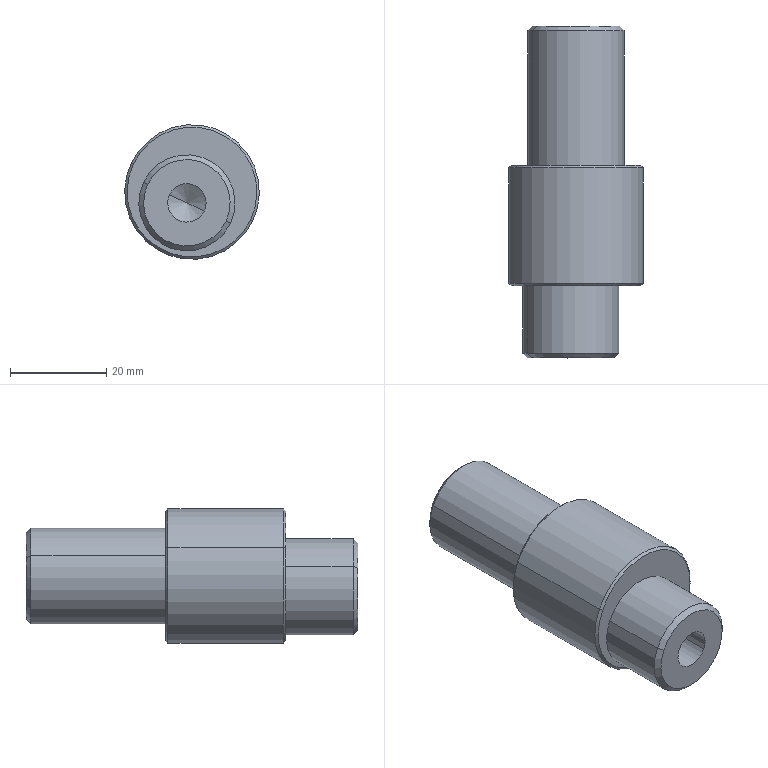Component | SolidWorks | Yk1.5.3RollerEccentricAxis-1 | 1 solid | 26 faces | box 28 x 69 x 28 mm | volume 27295 mm3 | cone 12 | cylinder 10 | plane 4 | commonest cylinder face diameters 8 x4 20 x4 28 x2 | material 45
build123d program:
from build123d import *

# Parameters (mm, degrees)
M8_TAPPED_HOLE2_D     = 8
M8_TAPPED_HOLE2_DEPTH = 15
M8_TAPPED_HOLE2_TIP   = 2.403
SKETCH4_R             = 10
BOSS_EXTRUDE1_DEPTH   = 15
CHAMFER1_SIZE         = 1
M8_TAPPED_HOLE1_D     = 8
M8_TAPPED_HOLE1_DEPTH = 20
M8_TAPPED_HOLE1_TIP   = 2.403
CHAMFER2_SIZE         = 0.5


with BuildPart() as part:
    # Sketch1 → Revolve1 (revolve)
    with BuildSketch(Plane.XY, mode=Mode.PRIVATE) as revolve1_sk:
        Polygon((14, 32.214), (0, 32.214), (0, 86.214), (10, 86.214), (10, 57.214), (14, 57.214), align=None)
    revolve(revolve1_sk.sketch.rotate(Axis((0, 0, 0), (0, 1, 0)), 90), axis=Axis((0, 0, 0), (0, 1, 0)))

    # M8 Tapped Hole2
    with Locations(Plane(origin=(0, 86.214, 0), x_dir=(1, 0, 0), z_dir=(0, 1, 0))):
        with Locations((0, 0)):
            Hole(M8_TAPPED_HOLE2_D / 2, depth=M8_TAPPED_HOLE2_DEPTH)
            with Locations((0, 0, -(M8_TAPPED_HOLE2_DEPTH + M8_TAPPED_HOLE2_TIP / 2))):  # 118° drill point
                Cone(0, M8_TAPPED_HOLE2_D / 2, M8_TAPPED_HOLE2_TIP, mode=Mode.SUBTRACT)

    # Sketch4 → Boss-Extrude1 (add)
    with BuildSketch(Plane(origin=(0, 32.214, 0), x_dir=(-1, 0, 0), z_dir=(0, -1, 0))):
        with Locations(Location((-2.5, 0, 0), (0, 0, 90))):
            Circle(SKETCH4_R)
    extrude(amount=BOSS_EXTRUDE1_DEPTH)

    # Chamfer1
    chamfer1_edges = [part.edges().sort_by_distance(p)[0] for p in [
        (2.5, 17.214, 10),
        (0, 86.214, 10),
    ]]
    chamfer(chamfer1_edges, length=CHAMFER1_SIZE)

    # M8 Tapped Hole1
    with Locations(Plane(origin=(0, 17.214, 0), x_dir=(-1, 0, 0), z_dir=(0, -1, 0))):
        with Locations((-2.5, 0)):
            Hole(M8_TAPPED_HOLE1_D / 2, depth=M8_TAPPED_HOLE1_DEPTH)
            with Locations((0, 0, -(M8_TAPPED_HOLE1_DEPTH + M8_TAPPED_HOLE1_TIP / 2))):  # 118° drill point
                Cone(0, M8_TAPPED_HOLE1_D / 2, M8_TAPPED_HOLE1_TIP, mode=Mode.SUBTRACT)

    # Chamfer2
    chamfer2_edges = [part.edges().sort_by_distance(p)[0] for p in [
        (0, 32.214, 14),
        (0, 57.214, 14),
    ]]
    chamfer(chamfer2_edges, length=CHAMFER2_SIZE)


solid = part.part

# Placed as in the assembly
solid = solid.moved(Location((-40.006, -57.214, 26), (180, 64.768, -180)))
STEP:
#1=COLOUR_RGB('',0.7922,0.8196,0.9333);
#2=FILL_AREA_STYLE_COLOUR('',#1);
#3=FILL_AREA_STYLE('',(#2));
#4=SURFACE_STYLE_FILL_AREA(#3);
#5=SURFACE_SIDE_STYLE('',(#4));
#6=SURFACE_STYLE_USAGE(.BOTH.,#5);
#7=PRESENTATION_STYLE_ASSIGNMENT((#6));
#8=CARTESIAN_POINT('',(-1.094,-0.,0.7971));
#9=VERTEX_POINT('',#8);
#10=CARTESIAN_POINT('',(-2.056,-0.,1.25));
#11=VERTEX_POINT('',#10);
#12=CARTESIAN_POINT('',(-1.575,-0.,1.024));
#13=DIRECTION('',(0.,1.,0.));
#14=DIRECTION('',(0.9046,0.,-0.4263));
#15=AXIS2_PLACEMENT_3D('',#12,#13,#14);
#16=CIRCLE('',#15,0.5315);
#17=EDGE_CURVE('',#9,#11,#16,.T.);
#18=ORIENTED_EDGE('',*,*,#17,.F.);
#19=CARTESIAN_POINT('',(-1.076,-0.01969,0.7887));
#20=VERTEX_POINT('',#19);
#21=CARTESIAN_POINT('',(-1.076,-0.01969,0.7887));
#22=DIRECTION('',(0.6396,-0.7071,-0.3014));
#23=VECTOR('',#22,39.37);
#24=LINE('',#21,#23);
#25=EDGE_CURVE('',#9,#20,#24,.T.);
#26=ORIENTED_EDGE('',*,*,#25,.T.);
#27=CARTESIAN_POINT('',(-2.074,-0.01969,1.259));
#28=VERTEX_POINT('',#27);
#29=CARTESIAN_POINT('',(-1.575,-0.01969,1.024));
#30=DIRECTION('',(0.,-1.,0.));
#31=DIRECTION('',(0.9046,0.,-0.4263));
#32=AXIS2_PLACEMENT_3D('',#29,#30,#31);
#33=CIRCLE('',#32,0.5512);
#34=EDGE_CURVE('',#28,#20,#33,.T.);
#35=ORIENTED_EDGE('',*,*,#34,.F.);
#36=CARTESIAN_POINT('',(-2.074,-0.01969,1.259));
#37=DIRECTION('',(-0.6396,-0.7071,0.3014));
#38=VECTOR('',#37,39.37);
#39=LINE('',#36,#38);
#40=EDGE_CURVE('',#11,#28,#39,.T.);
#41=ORIENTED_EDGE('',*,*,#40,.F.);
#42=EDGE_LOOP('',(#18,#26,#35,#41));
#43=FACE_OUTER_BOUND('',#42,.T.);
#44=CARTESIAN_POINT('',(-1.575,-0.01969,1.024));
#45=DIRECTION('',(0.,-1.,0.));
#46=DIRECTION('',(-0.9046,0.,0.4263));
#47=AXIS2_PLACEMENT_3D('',#44,#45,#46);
#48=CONICAL_SURFACE('',#47,0.5512,0.7854);
#49=ADVANCED_FACE('',(#43),#48,.T.);
#50=CARTESIAN_POINT('',(-2.056,-0.9843,1.25));
#51=VERTEX_POINT('',#50);
#52=CARTESIAN_POINT('',(-1.094,-0.9843,0.7971));
#53=VERTEX_POINT('',#52);
#54=CARTESIAN_POINT('',(-1.575,-0.9843,1.024));
#55=DIRECTION('',(0.,-1.,0.));
#56=DIRECTION('',(-0.9046,0.,0.4263));
#57=AXIS2_PLACEMENT_3D('',#54,#55,#56);
#58=CIRCLE('',#57,0.5315);
#59=EDGE_CURVE('',#51,#53,#58,.T.);
#60=ORIENTED_EDGE('',*,*,#59,.F.);
#61=CARTESIAN_POINT('',(-2.074,-0.9646,1.259));
#62=VERTEX_POINT('',#61);
#63=CARTESIAN_POINT('',(-2.056,-0.9843,1.25));
#64=DIRECTION('',(-0.6396,0.7071,0.3014));
#65=VECTOR('',#64,39.37);
#66=LINE('',#63,#65);
#67=EDGE_CURVE('',#51,#62,#66,.T.);
#68=ORIENTED_EDGE('',*,*,#67,.T.);
#69=CARTESIAN_POINT('',(-1.076,-0.9646,0.7887));
#70=VERTEX_POINT('',#69);
#71=CARTESIAN_POINT('',(-1.575,-0.9646,1.024));
#72=DIRECTION('',(0.,1.,0.));
#73=DIRECTION('',(-0.9046,0.,0.4263));
#74=AXIS2_PLACEMENT_3D('',#71,#72,#73);
#75=CIRCLE('',#74,0.5512);
#76=EDGE_CURVE('',#70,#62,#75,.T.);
#77=ORIENTED_EDGE('',*,*,#76,.F.);
#78=CARTESIAN_POINT('',(-1.094,-0.9843,0.7971));
#79=DIRECTION('',(0.6396,0.7071,-0.3014));
#80=VECTOR('',#79,39.37);
#81=LINE('',#78,#80);
#82=EDGE_CURVE('',#53,#70,#81,.T.);
#83=ORIENTED_EDGE('',*,*,#82,.F.);
#84=EDGE_LOOP('',(#60,#68,#77,#83));
#85=FACE_OUTER_BOUND('',#84,.T.);
#86=CARTESIAN_POINT('',(-1.575,-0.9843,1.024));
#87=DIRECTION('',(0.,1.,0.));
#88=DIRECTION('',(0.9046,0.,-0.4263));
#89=AXIS2_PLACEMENT_3D('',#86,#87,#88);
#90=CONICAL_SURFACE('',#89,0.5315,0.7854);
#91=ADVANCED_FACE('',(#85),#90,.T.);
#92=CARTESIAN_POINT('',(-1.475,-0.7874,0.8675));
#93=VERTEX_POINT('',#92);
#94=CARTESIAN_POINT('',(-1.759,-0.7874,1.002));
#95=VERTEX_POINT('',#94);
#96=CARTESIAN_POINT('',(-1.617,-0.7874,0.9346));
#97=DIRECTION('',(0.,-1.,0.));
#98=DIRECTION('',(-0.9046,0.,0.4263));
#99=AXIS2_PLACEMENT_3D('',#96,#97,#98);
#100=CIRCLE('',#99,0.1575);
#101=EDGE_CURVE('',#93,#95,#100,.T.);
#102=ORIENTED_EDGE('',*,*,#101,.F.);
#103=CARTESIAN_POINT('',(-1.475,-1.575,0.8675));
#104=VERTEX_POINT('',#103);
#105=CARTESIAN_POINT('',(-1.475,-1.575,0.8675));
#106=DIRECTION('',(0.,-1.,0.));
#107=VECTOR('',#106,39.37);
#108=LINE('',#105,#107);
#109=EDGE_CURVE('',#93,#104,#108,.T.);
#110=ORIENTED_EDGE('',*,*,#109,.T.);
#111=CARTESIAN_POINT('',(-1.759,-1.575,1.002));
#112=VERTEX_POINT('',#111);
#113=CARTESIAN_POINT('',(-1.617,-1.575,0.9346));
#114=DIRECTION('',(0.,-1.,0.));
#115=DIRECTION('',(-0.9046,0.,0.4263));
#116=AXIS2_PLACEMENT_3D('',#113,#114,#115);
#117=CIRCLE('',#116,0.1575);
#118=EDGE_CURVE('',#104,#112,#117,.T.);
#119=ORIENTED_EDGE('',*,*,#118,.T.);
#120=CARTESIAN_POINT('',(-1.759,-1.575,1.002));
#121=DIRECTION('',(0.,-1.,0.));
#122=VECTOR('',#121,39.37);
#123=LINE('',#120,#122);
#124=EDGE_CURVE('',#95,#112,#123,.T.);
#125=ORIENTED_EDGE('',*,*,#124,.F.);
#126=EDGE_LOOP('',(#102,#110,#119,#125));
#127=FACE_OUTER_BOUND('',#126,.T.);
#128=CARTESIAN_POINT('',(-1.617,-1.575,0.9346));
#129=DIRECTION('',(0.,-1.,0.));
#130=DIRECTION('',(-0.9046,0.,0.4263));
#131=AXIS2_PLACEMENT_3D('',#128,#129,#130);
#132=CYLINDRICAL_SURFACE('',#131,0.1575);
#133=ADVANCED_FACE('',(#127),#132,.F.);
#134=CARTESIAN_POINT('',(-1.617,-0.6928,0.9346));
#135=VERTEX_POINT('',#134);
#136=CARTESIAN_POINT('',(-1.759,-0.7874,1.002));
#137=DIRECTION('',(-0.7754,-0.515,0.3654));
#138=VECTOR('',#137,39.37);
#139=LINE('',#136,#138);
#140=EDGE_CURVE('',#135,#95,#139,.T.);
#141=ORIENTED_EDGE('',*,*,#140,.F.);
#142=CARTESIAN_POINT('',(-1.475,-0.7874,0.8675));
#143=DIRECTION('',(0.7754,-0.515,-0.3654));
#144=VECTOR('',#143,39.37);
#145=LINE('',#142,#144);
#146=EDGE_CURVE('',#135,#93,#145,.T.);
#147=ORIENTED_EDGE('',*,*,#146,.T.);
#148=ORIENTED_EDGE('',*,*,#101,.T.);
#149=EDGE_LOOP('',(#141,#147,#148));
#150=FACE_OUTER_BOUND('',#149,.T.);
#151=CARTESIAN_POINT('',(-1.617,-0.7874,0.9346));
#152=DIRECTION('',(0.,-1.,0.));
#153=DIRECTION('',(-0.9046,0.,0.4263));
#154=AXIS2_PLACEMENT_3D('',#151,#152,#153);
#155=CONICAL_SURFACE('',#154,0.1575,1.03);
#156=ADVANCED_FACE('',(#150),#155,.F.);
#157=CARTESIAN_POINT('',(-1.255,1.142,0.8726));
#158=VERTEX_POINT('',#157);
#159=CARTESIAN_POINT('',(-1.896,1.142,1.175));
#160=VERTEX_POINT('',#159);
#161=CARTESIAN_POINT('',(-1.575,1.142,1.024));
#162=DIRECTION('',(0.,1.,0.));
#163=DIRECTION('',(0.9046,0.,-0.4263));
#164=AXIS2_PLACEMENT_3D('',#161,#162,#163);
#165=CIRCLE('',#164,0.3543);
#166=EDGE_CURVE('',#158,#160,#165,.T.);
#167=ORIENTED_EDGE('',*,*,#166,.F.);
#168=CARTESIAN_POINT('',(-1.219,1.102,0.8558));
#169=VERTEX_POINT('',#168);
#170=CARTESIAN_POINT('',(-1.219,1.102,0.8558));
#171=DIRECTION('',(0.6396,-0.7071,-0.3014));
#172=VECTOR('',#171,39.37);
#173=LINE('',#170,#172);
#174=EDGE_CURVE('',#158,#169,#173,.T.);
#175=ORIENTED_EDGE('',*,*,#174,.T.);
#176=CARTESIAN_POINT('',(-1.931,1.102,1.191));
#177=VERTEX_POINT('',#176);
#178=CARTESIAN_POINT('',(-1.575,1.102,1.024));
#179=DIRECTION('',(0.,-1.,0.));
#180=DIRECTION('',(0.9046,0.,-0.4263));
#181=AXIS2_PLACEMENT_3D('',#178,#179,#180);
#182=CIRCLE('',#181,0.3937);
#183=EDGE_CURVE('',#177,#169,#182,.T.);
#184=ORIENTED_EDGE('',*,*,#183,.F.);
#185=CARTESIAN_POINT('',(-1.931,1.102,1.191));
#186=DIRECTION('',(-0.6396,-0.7071,0.3014));
#187=VECTOR('',#186,39.37);
#188=LINE('',#185,#187);
#189=EDGE_CURVE('',#160,#177,#188,.T.);
#190=ORIENTED_EDGE('',*,*,#189,.F.);
#191=EDGE_LOOP('',(#167,#175,#184,#190));
#192=FACE_OUTER_BOUND('',#191,.T.);
#193=CARTESIAN_POINT('',(-1.575,1.102,1.024));
#194=DIRECTION('',(0.,-1.,0.));
#195=DIRECTION('',(-0.9046,0.,0.4263));
#196=AXIS2_PLACEMENT_3D('',#193,#194,#195);
#197=CONICAL_SURFACE('',#196,0.3937,0.7854);
#198=ADVANCED_FACE('',(#192),#197,.T.);
#199=CARTESIAN_POINT('',(-1.938,-1.575,1.086));
#200=VERTEX_POINT('',#199);
#201=CARTESIAN_POINT('',(-1.296,-1.575,0.7835));
#202=VERTEX_POINT('',#201);
#203=CARTESIAN_POINT('',(-1.617,-1.575,0.9346));
#204=DIRECTION('',(0.,-1.,0.));
#205=DIRECTION('',(-0.9046,0.,0.4263));
#206=AXIS2_PLACEMENT_3D('',#203,#204,#205);
#207=CIRCLE('',#206,0.3543);
#208=EDGE_CURVE('',#200,#202,#207,.T.);
#209=ORIENTED_EDGE('',*,*,#208,.F.);
#210=CARTESIAN_POINT('',(-1.973,-1.535,1.102));
#211=VERTEX_POINT('',#210);
#212=CARTESIAN_POINT('',(-1.938,-1.575,1.086));
#213=DIRECTION('',(-0.6396,0.7071,0.3014));
#214=VECTOR('',#213,39.37);
#215=LINE('',#212,#214);
#216=EDGE_CURVE('',#200,#211,#215,.T.);
#217=ORIENTED_EDGE('',*,*,#216,.T.);
#218=CARTESIAN_POINT('',(-1.261,-1.535,0.7668));
#219=VERTEX_POINT('',#218);
#220=CARTESIAN_POINT('',(-1.617,-1.535,0.9346));
#221=DIRECTION('',(0.,1.,0.));
#222=DIRECTION('',(-0.9046,0.,0.4263));
#223=AXIS2_PLACEMENT_3D('',#220,#221,#222);
#224=CIRCLE('',#223,0.3937);
#225=EDGE_CURVE('',#219,#211,#224,.T.);
#226=ORIENTED_EDGE('',*,*,#225,.F.);
#227=CARTESIAN_POINT('',(-1.296,-1.575,0.7835));
#228=DIRECTION('',(0.6396,0.7071,-0.3014));
#229=VECTOR('',#228,39.37);
#230=LINE('',#227,#229);
#231=EDGE_CURVE('',#202,#219,#230,.T.);
#232=ORIENTED_EDGE('',*,*,#231,.F.);
#233=EDGE_LOOP('',(#209,#217,#226,#232));
#234=FACE_OUTER_BOUND('',#233,.T.);
#235=CARTESIAN_POINT('',(-1.617,-1.575,0.9346));
#236=DIRECTION('',(0.,1.,0.));
#237=DIRECTION('',(0.9046,0.,-0.4263));
#238=AXIS2_PLACEMENT_3D('',#235,#236,#237);
#239=CONICAL_SURFACE('',#238,0.3543,0.7854);
#240=ADVANCED_FACE('',(#234),#239,.T.);
#241=ORIENTED_EDGE('',*,*,#225,.T.);
#242=CARTESIAN_POINT('',(-1.973,-0.9843,1.102));
#243=VERTEX_POINT('',#242);
#244=CARTESIAN_POINT('',(-1.973,-1.575,1.102));
#245=DIRECTION('',(0.,1.,0.));
#246=VECTOR('',#245,39.37);
#247=LINE('',#244,#246);
#248=EDGE_CURVE('',#211,#243,#247,.T.);
#249=ORIENTED_EDGE('',*,*,#248,.T.);
#250=CARTESIAN_POINT('',(-1.261,-0.9843,0.7668));
#251=VERTEX_POINT('',#250);
#252=CARTESIAN_POINT('',(-1.617,-0.9843,0.9346));
#253=DIRECTION('',(0.,-1.,0.));
#254=DIRECTION('',(-0.9046,0.,0.4263));
#255=AXIS2_PLACEMENT_3D('',#252,#253,#254);
#256=CIRCLE('',#255,0.3937);
#257=EDGE_CURVE('',#243,#251,#256,.T.);
#258=ORIENTED_EDGE('',*,*,#257,.T.);
#259=CARTESIAN_POINT('',(-1.261,-1.575,0.7668));
#260=DIRECTION('',(0.,1.,0.));
#261=VECTOR('',#260,39.37);
#262=LINE('',#259,#261);
#263=EDGE_CURVE('',#219,#251,#262,.T.);
#264=ORIENTED_EDGE('',*,*,#263,.F.);
#265=EDGE_LOOP('',(#241,#249,#258,#264));
#266=FACE_OUTER_BOUND('',#265,.T.);
#267=CARTESIAN_POINT('',(-1.617,-1.575,0.9346));
#268=DIRECTION('',(0.,1.,0.));
#269=DIRECTION('',(0.9046,0.,-0.4263));
#270=AXIS2_PLACEMENT_3D('',#267,#268,#269);
#271=CYLINDRICAL_SURFACE('',#270,0.3937);
#272=ADVANCED_FACE('',(#266),#271,.T.);
#273=CARTESIAN_POINT('',(-1.718,0.5512,1.091));
#274=VERTEX_POINT('',#273);
#275=CARTESIAN_POINT('',(-1.433,0.5512,0.9565));
#276=VERTEX_POINT('',#275);
#277=CARTESIAN_POINT('',(-1.575,0.5512,1.024));
#278=DIRECTION('',(0.,1.,0.));
#279=DIRECTION('',(0.9046,0.,-0.4263));
#280=AXIS2_PLACEMENT_3D('',#277,#278,#279);
#281=CIRCLE('',#280,0.1575);
#282=EDGE_CURVE('',#274,#276,#281,.T.);
#283=ORIENTED_EDGE('',*,*,#282,.F.);
#284=CARTESIAN_POINT('',(-1.718,1.142,1.091));
#285=VERTEX_POINT('',#284);
#286=CARTESIAN_POINT('',(-1.718,1.142,1.091));
#287=DIRECTION('',(0.,1.,0.));
#288=VECTOR('',#287,39.37);
#289=LINE('',#286,#288);
#290=EDGE_CURVE('',#274,#285,#289,.T.);
#291=ORIENTED_EDGE('',*,*,#290,.T.);
#292=CARTESIAN_POINT('',(-1.433,1.142,0.9565));
#293=VERTEX_POINT('',#292);
#294=CARTESIAN_POINT('',(-1.575,1.142,1.024));
#295=DIRECTION('',(0.,1.,0.));
#296=DIRECTION('',(0.9046,0.,-0.4263));
#297=AXIS2_PLACEMENT_3D('',#294,#295,#296);
#298=CIRCLE('',#297,0.1575);
#299=EDGE_CURVE('',#285,#293,#298,.T.);
#300=ORIENTED_EDGE('',*,*,#299,.T.);
#301=CARTESIAN_POINT('',(-1.433,1.142,0.9565));
#302=DIRECTION('',(0.,1.,0.));
#303=VECTOR('',#302,39.37);
#304=LINE('',#301,#303);
#305=EDGE_CURVE('',#276,#293,#304,.T.);
#306=ORIENTED_EDGE('',*,*,#305,.F.);
#307=EDGE_LOOP('',(#283,#291,#300,#306));
#308=FACE_OUTER_BOUND('',#307,.T.);
#309=CARTESIAN_POINT('',(-1.575,1.142,1.024));
#310=DIRECTION('',(0.,1.,0.));
#311=DIRECTION('',(0.9046,0.,-0.4263));
#312=AXIS2_PLACEMENT_3D('',#309,#310,#311);
#313=CYLINDRICAL_SURFACE('',#312,0.1575);
#314=ADVANCED_FACE('',(#308),#313,.F.);
#315=CARTESIAN_POINT('',(-1.575,0.4566,1.024));
#316=VERTEX_POINT('',#315);
#317=CARTESIAN_POINT('',(-1.433,0.5512,0.9565));
#318=DIRECTION('',(0.7754,0.515,-0.3654));
#319=VECTOR('',#318,39.37);
#320=LINE('',#317,#319);
#321=EDGE_CURVE('',#316,#276,#320,.T.);
#322=ORIENTED_EDGE('',*,*,#321,.F.);
#323=CARTESIAN_POINT('',(-1.718,0.5512,1.091));
#324=DIRECTION('',(-0.7754,0.515,0.3654));
#325=VECTOR('',#324,39.37);
#326=LINE('',#323,#325);
#327=EDGE_CURVE('',#316,#274,#326,.T.);
#328=ORIENTED_EDGE('',*,*,#327,.T.);
#329=ORIENTED_EDGE('',*,*,#282,.T.);
#330=EDGE_LOOP('',(#322,#328,#329));
#331=FACE_OUTER_BOUND('',#330,.T.);
#332=CARTESIAN_POINT('',(-1.575,0.5512,1.024));
#333=DIRECTION('',(0.,1.,0.));
#334=DIRECTION('',(0.9046,0.,-0.4263));
#335=AXIS2_PLACEMENT_3D('',#332,#333,#334);
#336=CONICAL_SURFACE('',#335,0.1575,1.03);
#337=ADVANCED_FACE('',(#331),#336,.F.);
#338=ORIENTED_EDGE('',*,*,#34,.T.);
#339=CARTESIAN_POINT('',(-1.076,-2.253,0.7887));
#340=DIRECTION('',(0.,-1.,0.));
#341=VECTOR('',#340,39.37);
#342=LINE('',#339,#341);
#343=EDGE_CURVE('',#20,#70,#342,.T.);
#344=ORIENTED_EDGE('',*,*,#343,.T.);
#345=ORIENTED_EDGE('',*,*,#76,.T.);
#346=CARTESIAN_POINT('',(-2.074,-2.253,1.259));
#347=DIRECTION('',(0.,-1.,0.));
#348=VECTOR('',#347,39.37);
#349=LINE('',#346,#348);
#350=EDGE_CURVE('',#28,#62,#349,.T.);
#351=ORIENTED_EDGE('',*,*,#350,.F.);
#352=EDGE_LOOP('',(#338,#344,#345,#351));
#353=FACE_OUTER_BOUND('',#352,.T.);
#354=CARTESIAN_POINT('',(-1.575,-2.253,1.024));
#355=DIRECTION('',(0.,-1.,0.));
#356=DIRECTION('',(-0.9046,0.,0.4263));
#357=AXIS2_PLACEMENT_3D('',#354,#355,#356);
#358=CYLINDRICAL_SURFACE('',#357,0.5512);
#359=ADVANCED_FACE('',(#353),#358,.T.);
#360=ORIENTED_EDGE('',*,*,#183,.T.);
#361=CARTESIAN_POINT('',(-1.219,-0.,0.8558));
#362=VERTEX_POINT('',#361);
#363=CARTESIAN_POINT('',(-1.219,-2.253,0.8558));
#364=DIRECTION('',(0.,-1.,0.));
#365=VECTOR('',#364,39.37);
#366=LINE('',#363,#365);
#367=EDGE_CURVE('',#169,#362,#366,.T.);
#368=ORIENTED_EDGE('',*,*,#367,.T.);
#369=CARTESIAN_POINT('',(-1.931,-0.,1.191));
#370=VERTEX_POINT('',#369);
#371=CARTESIAN_POINT('',(-1.575,-0.,1.024));
#372=DIRECTION('',(0.,-1.,0.));
#373=DIRECTION('',(-0.9046,0.,0.4263));
#374=AXIS2_PLACEMENT_3D('',#371,#372,#373);
#375=CIRCLE('',#374,0.3937);
#376=EDGE_CURVE('',#370,#362,#375,.T.);
#377=ORIENTED_EDGE('',*,*,#376,.F.);
#378=CARTESIAN_POINT('',(-1.931,-2.253,1.191));
#379=DIRECTION('',(0.,-1.,0.));
#380=VECTOR('',#379,39.37);
#381=LINE('',#378,#380);
#382=EDGE_CURVE('',#177,#370,#381,.T.);
#383=ORIENTED_EDGE('',*,*,#382,.F.);
#384=EDGE_LOOP('',(#360,#368,#377,#383));
#385=FACE_OUTER_BOUND('',#384,.T.);
#386=CARTESIAN_POINT('',(-1.575,-2.253,1.024));
#387=DIRECTION('',(0.,-1.,0.));
#388=DIRECTION('',(-0.9046,0.,0.4263));
#389=AXIS2_PLACEMENT_3D('',#386,#387,#388);
#390=CYLINDRICAL_SURFACE('',#389,0.3937);
#391=ADVANCED_FACE('',(#385),#390,.T.);
#392=CARTESIAN_POINT('',(-1.575,-0.9843,1.024));
#393=DIRECTION('',(0.,-1.,0.));
#394=DIRECTION('',(-0.9046,0.,0.4263));
#395=AXIS2_PLACEMENT_3D('',#392,#393,#394);
#396=CIRCLE('',#395,0.5315);
#397=EDGE_CURVE('',#53,#51,#396,.T.);
#398=ORIENTED_EDGE('',*,*,#397,.T.);
#399=ORIENTED_EDGE('',*,*,#59,.T.);
#400=EDGE_LOOP('',(#398,#399));
#401=FACE_OUTER_BOUND('',#400,.T.);
#402=CARTESIAN_POINT('',(-1.617,-0.9843,0.9346));
#403=DIRECTION('',(0.,-1.,0.));
#404=DIRECTION('',(-0.9046,0.,0.4263));
#405=AXIS2_PLACEMENT_3D('',#402,#403,#404);
#406=CIRCLE('',#405,0.3937);
#407=EDGE_CURVE('',#251,#243,#406,.T.);
#408=ORIENTED_EDGE('',*,*,#407,.F.);
#409=ORIENTED_EDGE('',*,*,#257,.F.);
#410=EDGE_LOOP('',(#408,#409));
#411=FACE_BOUND('',#410,.T.);
#412=CARTESIAN_POINT('',(-1.81,-0.9843,0.525));
#413=DIRECTION('',(0.,-1.,0.));
#414=DIRECTION('',(-0.9046,0.,0.4263));
#415=AXIS2_PLACEMENT_3D('',#412,#413,#414);
#416=PLANE('',#415);
#417=ADVANCED_FACE('',(#401,#411),#416,.T.);
#418=CARTESIAN_POINT('',(-1.575,1.142,1.024));
#419=DIRECTION('',(0.,1.,0.));
#420=DIRECTION('',(0.9046,0.,-0.4263));
#421=AXIS2_PLACEMENT_3D('',#418,#419,#420);
#422=CIRCLE('',#421,0.3543);
#423=EDGE_CURVE('',#160,#158,#422,.T.);
#424=ORIENTED_EDGE('',*,*,#423,.T.);
#425=ORIENTED_EDGE('',*,*,#166,.T.);
#426=EDGE_LOOP('',(#424,#425));
#427=FACE_OUTER_BOUND('',#426,.T.);
#428=CARTESIAN_POINT('',(-1.575,1.142,1.024));
#429=DIRECTION('',(0.,1.,0.));
#430=DIRECTION('',(0.9046,0.,-0.4263));
#431=AXIS2_PLACEMENT_3D('',#428,#429,#430);
#432=CIRCLE('',#431,0.1575);
#433=EDGE_CURVE('',#293,#285,#432,.T.);
#434=ORIENTED_EDGE('',*,*,#433,.F.);
#435=ORIENTED_EDGE('',*,*,#299,.F.);
#436=EDGE_LOOP('',(#434,#435));
#437=FACE_BOUND('',#436,.T.);
#438=CARTESIAN_POINT('',(-1.575,1.142,1.024));
#439=DIRECTION('',(0.,1.,0.));
#440=DIRECTION('',(0.9046,0.,-0.4263));
#441=AXIS2_PLACEMENT_3D('',#438,#439,#440);
#442=PLANE('',#441);
#443=ADVANCED_FACE('',(#427,#437),#442,.T.);
#444=ORIENTED_EDGE('',*,*,#367,.F.);
#445=CARTESIAN_POINT('',(-1.575,1.102,1.024));
#446=DIRECTION('',(0.,-1.,0.));
#447=DIRECTION('',(0.9046,0.,-0.4263));
#448=AXIS2_PLACEMENT_3D('',#445,#446,#447);
#449=CIRCLE('',#448,0.3937);
#450=EDGE_CURVE('',#169,#177,#449,.T.);
#451=ORIENTED_EDGE('',*,*,#450,.T.);
#452=ORIENTED_EDGE('',*,*,#382,.T.);
#453=CARTESIAN_POINT('',(-1.575,-0.,1.024));
#454=DIRECTION('',(0.,-1.,0.));
#455=DIRECTION('',(-0.9046,0.,0.4263));
#456=AXIS2_PLACEMENT_3D('',#453,#454,#455);
#457=CIRCLE('',#456,0.3937);
#458=EDGE_CURVE('',#362,#370,#457,.T.);
#459=ORIENTED_EDGE('',*,*,#458,.F.);
#460=EDGE_LOOP('',(#444,#451,#452,#459));
#461=FACE_OUTER_BOUND('',#460,.T.);
#462=CARTESIAN_POINT('',(-1.575,-2.253,1.024));
#463=DIRECTION('',(0.,-1.,0.));
#464=DIRECTION('',(-0.9046,0.,0.4263));
#465=AXIS2_PLACEMENT_3D('',#462,#463,#464);
#466=CYLINDRICAL_SURFACE('',#465,0.3937);
#467=ADVANCED_FACE('',(#461),#466,.T.);
#468=CARTESIAN_POINT('',(-1.575,-0.,1.024));
#469=DIRECTION('',(0.,1.,0.));
#470=DIRECTION('',(0.9046,0.,-0.4263));
#471=AXIS2_PLACEMENT_3D('',#468,#469,#470);
#472=CIRCLE('',#471,0.5315);
#473=EDGE_CURVE('',#11,#9,#472,.T.);
#474=ORIENTED_EDGE('',*,*,#473,.T.);
#475=ORIENTED_EDGE('',*,*,#17,.T.);
#476=EDGE_LOOP('',(#474,#475));
#477=FACE_OUTER_BOUND('',#476,.T.);
#478=ORIENTED_EDGE('',*,*,#376,.T.);
#479=ORIENTED_EDGE('',*,*,#458,.T.);
#480=EDGE_LOOP('',(#478,#479));
#481=FACE_BOUND('',#480,.T.);
#482=CARTESIAN_POINT('',(-1.743,-0.,0.6675));
#483=DIRECTION('',(0.,1.,0.));
#484=DIRECTION('',(0.9046,0.,-0.4263));
#485=AXIS2_PLACEMENT_3D('',#482,#483,#484);
#486=PLANE('',#485);
#487=ADVANCED_FACE('',(#477,#481),#486,.T.);
#488=ORIENTED_EDGE('',*,*,#343,.F.);
#489=CARTESIAN_POINT('',(-1.575,-0.01969,1.024));
#490=DIRECTION('',(0.,-1.,0.));
#491=DIRECTION('',(0.9046,0.,-0.4263));
#492=AXIS2_PLACEMENT_3D('',#489,#490,#491);
#493=CIRCLE('',#492,0.5512);
#494=EDGE_CURVE('',#20,#28,#493,.T.);
#495=ORIENTED_EDGE('',*,*,#494,.T.);
#496=ORIENTED_EDGE('',*,*,#350,.T.);
#497=CARTESIAN_POINT('',(-1.575,-0.9646,1.024));
#498=DIRECTION('',(0.,1.,0.));
#499=DIRECTION('',(-0.9046,0.,0.4263));
#500=AXIS2_PLACEMENT_3D('',#497,#498,#499);
#501=CIRCLE('',#500,0.5512);
#502=EDGE_CURVE('',#62,#70,#501,.T.);
#503=ORIENTED_EDGE('',*,*,#502,.T.);
#504=EDGE_LOOP('',(#488,#495,#496,#503));
#505=FACE_OUTER_BOUND('',#504,.T.);
#506=CARTESIAN_POINT('',(-1.575,-2.253,1.024));
#507=DIRECTION('',(0.,-1.,0.));
#508=DIRECTION('',(-0.9046,0.,0.4263));
#509=AXIS2_PLACEMENT_3D('',#506,#507,#508);
#510=CYLINDRICAL_SURFACE('',#509,0.5512);
#511=ADVANCED_FACE('',(#505),#510,.T.);
#512=ORIENTED_EDGE('',*,*,#327,.F.);
#513=ORIENTED_EDGE('',*,*,#321,.T.);
#514=CARTESIAN_POINT('',(-1.575,0.5512,1.024));
#515=DIRECTION('',(0.,1.,0.));
#516=DIRECTION('',(0.9046,0.,-0.4263));
#517=AXIS2_PLACEMENT_3D('',#514,#515,#516);
#518=CIRCLE('',#517,0.1575);
#519=EDGE_CURVE('',#276,#274,#518,.T.);
#520=ORIENTED_EDGE('',*,*,#519,.T.);
#521=EDGE_LOOP('',(#512,#513,#520));
#522=FACE_OUTER_BOUND('',#521,.T.);
#523=CARTESIAN_POINT('',(-1.575,0.5512,1.024));
#524=DIRECTION('',(0.,1.,0.));
#525=DIRECTION('',(0.9046,0.,-0.4263));
#526=AXIS2_PLACEMENT_3D('',#523,#524,#525);
#527=CONICAL_SURFACE('',#526,0.1575,1.03);
#528=ADVANCED_FACE('',(#522),#527,.F.);
#529=ORIENTED_EDGE('',*,*,#290,.F.);
#530=ORIENTED_EDGE('',*,*,#519,.F.);
#531=ORIENTED_EDGE('',*,*,#305,.T.);
#532=ORIENTED_EDGE('',*,*,#433,.T.);
#533=EDGE_LOOP('',(#529,#530,#531,#532));
#534=FACE_OUTER_BOUND('',#533,.T.);
#535=CARTESIAN_POINT('',(-1.575,1.142,1.024));
#536=DIRECTION('',(0.,1.,0.));
#537=DIRECTION('',(0.9046,0.,-0.4263));
#538=AXIS2_PLACEMENT_3D('',#535,#536,#537);
#539=CYLINDRICAL_SURFACE('',#538,0.1575);
#540=ADVANCED_FACE('',(#534),#539,.F.);
#541=ORIENTED_EDGE('',*,*,#248,.F.);
#542=CARTESIAN_POINT('',(-1.617,-1.535,0.9346));
#543=DIRECTION('',(0.,1.,0.));
#544=DIRECTION('',(-0.9046,0.,0.4263));
#545=AXIS2_PLACEMENT_3D('',#542,#543,#544);
#546=CIRCLE('',#545,0.3937);
#547=EDGE_CURVE('',#211,#219,#546,.T.);
#548=ORIENTED_EDGE('',*,*,#547,.T.);
#549=ORIENTED_EDGE('',*,*,#263,.T.);
#550=ORIENTED_EDGE('',*,*,#407,.T.);
#551=EDGE_LOOP('',(#541,#548,#549,#550));
#552=FACE_OUTER_BOUND('',#551,.T.);
#553=CARTESIAN_POINT('',(-1.617,-1.575,0.9346));
#554=DIRECTION('',(0.,1.,0.));
#555=DIRECTION('',(0.9046,0.,-0.4263));
#556=AXIS2_PLACEMENT_3D('',#553,#554,#555);
#557=CYLINDRICAL_SURFACE('',#556,0.3937);
#558=ADVANCED_FACE('',(#552),#557,.T.);
#559=CARTESIAN_POINT('',(-1.617,-1.575,0.9346));
#560=DIRECTION('',(0.,-1.,0.));
#561=DIRECTION('',(-0.9046,0.,0.4263));
#562=AXIS2_PLACEMENT_3D('',#559,#560,#561);
#563=CIRCLE('',#562,0.1575);
#564=EDGE_CURVE('',#112,#104,#563,.T.);
#565=ORIENTED_EDGE('',*,*,#564,.F.);
#566=ORIENTED_EDGE('',*,*,#118,.F.);
#567=EDGE_LOOP('',(#565,#566));
#568=FACE_BOUND('',#567,.T.);
#569=CARTESIAN_POINT('',(-1.617,-1.575,0.9346));
#570=DIRECTION('',(0.,-1.,0.));
#571=DIRECTION('',(-0.9046,0.,0.4263));
#572=AXIS2_PLACEMENT_3D('',#569,#570,#571);
#573=CIRCLE('',#572,0.3543);
#574=EDGE_CURVE('',#202,#200,#573,.T.);
#575=ORIENTED_EDGE('',*,*,#574,.T.);
#576=ORIENTED_EDGE('',*,*,#208,.T.);
#577=EDGE_LOOP('',(#575,#576));
#578=FACE_OUTER_BOUND('',#577,.T.);
#579=CARTESIAN_POINT('',(-1.617,-1.575,0.9346));
#580=DIRECTION('',(0.,-1.,0.));
#581=DIRECTION('',(-0.9046,0.,0.4263));
#582=AXIS2_PLACEMENT_3D('',#579,#580,#581);
#583=PLANE('',#582);
#584=ADVANCED_FACE('',(#568,#578),#583,.T.);
#585=ORIENTED_EDGE('',*,*,#216,.F.);
#586=ORIENTED_EDGE('',*,*,#574,.F.);
#587=ORIENTED_EDGE('',*,*,#231,.T.);
#588=ORIENTED_EDGE('',*,*,#547,.F.);
#589=EDGE_LOOP('',(#585,#586,#587,#588));
#590=FACE_OUTER_BOUND('',#589,.T.);
#591=CARTESIAN_POINT('',(-1.617,-1.575,0.9346));
#592=DIRECTION('',(0.,1.,0.));
#593=DIRECTION('',(0.9046,0.,-0.4263));
#594=AXIS2_PLACEMENT_3D('',#591,#592,#593);
#595=CONICAL_SURFACE('',#594,0.3543,0.7854);
#596=ADVANCED_FACE('',(#590),#595,.T.);
#597=ORIENTED_EDGE('',*,*,#174,.F.);
#598=ORIENTED_EDGE('',*,*,#423,.F.);
#599=ORIENTED_EDGE('',*,*,#189,.T.);
#600=ORIENTED_EDGE('',*,*,#450,.F.);
#601=EDGE_LOOP('',(#597,#598,#599,#600));
#602=FACE_OUTER_BOUND('',#601,.T.);
#603=CARTESIAN_POINT('',(-1.575,1.102,1.024));
#604=DIRECTION('',(0.,-1.,0.));
#605=DIRECTION('',(-0.9046,0.,0.4263));
#606=AXIS2_PLACEMENT_3D('',#603,#604,#605);
#607=CONICAL_SURFACE('',#606,0.3937,0.7854);
#608=ADVANCED_FACE('',(#602),#607,.T.);
#609=ORIENTED_EDGE('',*,*,#146,.F.);
#610=ORIENTED_EDGE('',*,*,#140,.T.);
#611=CARTESIAN_POINT('',(-1.617,-0.7874,0.9346));
#612=DIRECTION('',(0.,-1.,0.));
#613=DIRECTION('',(-0.9046,0.,0.4263));
#614=AXIS2_PLACEMENT_3D('',#611,#612,#613);
#615=CIRCLE('',#614,0.1575);
#616=EDGE_CURVE('',#95,#93,#615,.T.);
#617=ORIENTED_EDGE('',*,*,#616,.T.);
#618=EDGE_LOOP('',(#609,#610,#617));
#619=FACE_OUTER_BOUND('',#618,.T.);
#620=CARTESIAN_POINT('',(-1.617,-0.7874,0.9346));
#621=DIRECTION('',(0.,-1.,0.));
#622=DIRECTION('',(-0.9046,0.,0.4263));
#623=AXIS2_PLACEMENT_3D('',#620,#621,#622);
#624=CONICAL_SURFACE('',#623,0.1575,1.03);
#625=ADVANCED_FACE('',(#619),#624,.F.);
#626=ORIENTED_EDGE('',*,*,#109,.F.);
#627=ORIENTED_EDGE('',*,*,#616,.F.);
#628=ORIENTED_EDGE('',*,*,#124,.T.);
#629=ORIENTED_EDGE('',*,*,#564,.T.);
#630=EDGE_LOOP('',(#626,#627,#628,#629));
#631=FACE_OUTER_BOUND('',#630,.T.);
#632=CARTESIAN_POINT('',(-1.617,-1.575,0.9346));
#633=DIRECTION('',(0.,-1.,0.));
#634=DIRECTION('',(-0.9046,0.,0.4263));
#635=AXIS2_PLACEMENT_3D('',#632,#633,#634);
#636=CYLINDRICAL_SURFACE('',#635,0.1575);
#637=ADVANCED_FACE('',(#631),#636,.F.);
#638=ORIENTED_EDGE('',*,*,#67,.F.);
#639=ORIENTED_EDGE('',*,*,#397,.F.);
#640=ORIENTED_EDGE('',*,*,#82,.T.);
#641=ORIENTED_EDGE('',*,*,#502,.F.);
#642=EDGE_LOOP('',(#638,#639,#640,#641));
#643=FACE_OUTER_BOUND('',#642,.T.);
#644=CARTESIAN_POINT('',(-1.575,-0.9843,1.024));
#645=DIRECTION('',(0.,1.,0.));
#646=DIRECTION('',(0.9046,0.,-0.4263));
#647=AXIS2_PLACEMENT_3D('',#644,#645,#646);
#648=CONICAL_SURFACE('',#647,0.5315,0.7854);
#649=ADVANCED_FACE('',(#643),#648,.T.);
#650=ORIENTED_EDGE('',*,*,#25,.F.);
#651=ORIENTED_EDGE('',*,*,#473,.F.);
#652=ORIENTED_EDGE('',*,*,#40,.T.);
#653=ORIENTED_EDGE('',*,*,#494,.F.);
#654=EDGE_LOOP('',(#650,#651,#652,#653));
#655=FACE_OUTER_BOUND('',#654,.T.);
#656=CARTESIAN_POINT('',(-1.575,-0.01969,1.024));
#657=DIRECTION('',(0.,-1.,0.));
#658=DIRECTION('',(-0.9046,0.,0.4263));
#659=AXIS2_PLACEMENT_3D('',#656,#657,#658);
#660=CONICAL_SURFACE('',#659,0.5512,0.7854);
#661=ADVANCED_FACE('',(#655),#660,.T.);
#662=CLOSED_SHELL('',(#49,#91,#133,#156,#198,#240,#272,#314,#337,#359,#391,#417,#443,#467,#487,#511,#528,#540,#558,#584,#596,#608,#625,#637,#649,#661));
#663=MANIFOLD_SOLID_BREP('',#662);
#664=STYLED_ITEM('',(#7),#663);
#665=PRESENTATION_LAYER_ASSIGNMENT('','',(#664));
#666=CARTESIAN_POINT('',(0.,0.,0.));
#667=DIRECTION('',(0.,0.,1.));
#668=DIRECTION('',(1.,0.,0.));
#669=AXIS2_PLACEMENT_3D('',#666,#667,#668);
#670=(LENGTH_UNIT()NAMED_UNIT(*)SI_UNIT($,.METRE.));
#671=LENGTH_MEASURE_WITH_UNIT(LENGTH_MEASURE(0.0254),#670);
#672=DIMENSIONAL_EXPONENTS(1.,0.,0.,0.,0.,0.,0.);
#673=(CONVERSION_BASED_UNIT('',#671)LENGTH_UNIT()NAMED_UNIT(#672));
#674=UNCERTAINTY_MEASURE_WITH_UNIT(LENGTH_MEASURE(0.00001),#673,'','');
#675=(NAMED_UNIT(*)PLANE_ANGLE_UNIT()SI_UNIT($,.RADIAN.));
#676=(NAMED_UNIT(*)SI_UNIT($,.STERADIAN.)SOLID_ANGLE_UNIT());
#677=(GEOMETRIC_REPRESENTATION_CONTEXT(3)GLOBAL_UNCERTAINTY_ASSIGNED_CONTEXT((#674))GLOBAL_UNIT_ASSIGNED_CONTEXT((#673,#675,#676))REPRESENTATION_CONTEXT('',''));
#678=ADVANCED_BREP_SHAPE_REPRESENTATION('',(#663,#669),#677);
#679=(LENGTH_UNIT()NAMED_UNIT(*)SI_UNIT($,.METRE.));
#680=LENGTH_MEASURE_WITH_UNIT(LENGTH_MEASURE(0.0254),#679);
#681=DIMENSIONAL_EXPONENTS(1.,0.,0.,0.,0.,0.,0.);
#682=(CONVERSION_BASED_UNIT('',#680)LENGTH_UNIT()NAMED_UNIT(#681));
#683=UNCERTAINTY_MEASURE_WITH_UNIT(LENGTH_MEASURE(0.00001),#682,'','');
#684=(NAMED_UNIT(*)PLANE_ANGLE_UNIT()SI_UNIT($,.RADIAN.));
#685=(NAMED_UNIT(*)SI_UNIT($,.STERADIAN.)SOLID_ANGLE_UNIT());
#686=(GEOMETRIC_REPRESENTATION_CONTEXT(3)GLOBAL_UNCERTAINTY_ASSIGNED_CONTEXT((#683))GLOBAL_UNIT_ASSIGNED_CONTEXT((#682,#684,#685))REPRESENTATION_CONTEXT('',''));
#687=MECHANICAL_DESIGN_GEOMETRIC_PRESENTATION_REPRESENTATION('',(#664),#686);